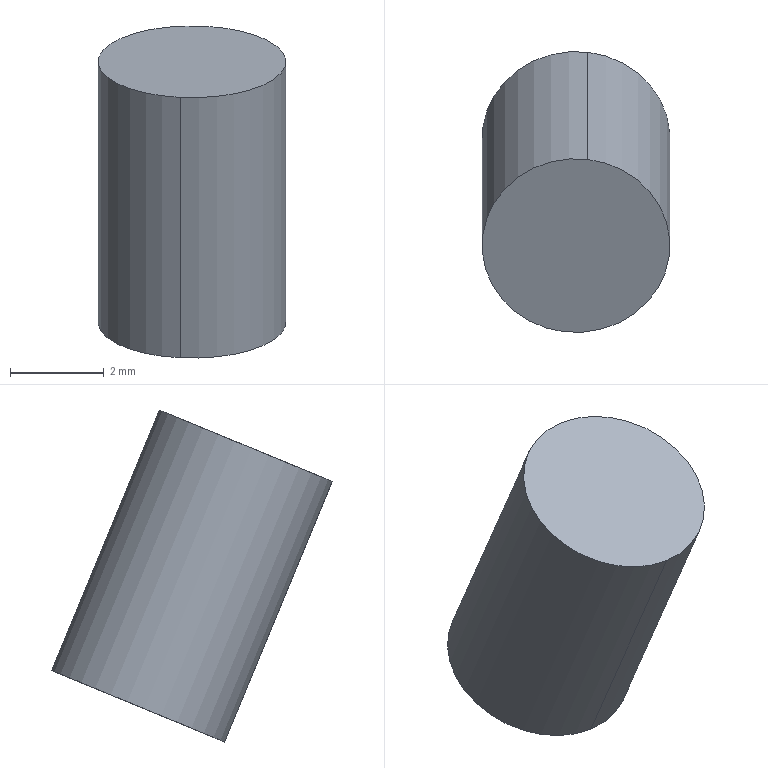Component | SolidWorks | Mirrorpin2-5 | 1 solid | 4 faces | box 4 x 5.99 x 7.07 mm | volume 75 mm3 | cylinder 2 | plane 2 | commonest cylinder face diameters 4 x2
STEP:
#1=COLOUR_RGB('',0.7922,0.8196,0.9333);
#2=FILL_AREA_STYLE_COLOUR('',#1);
#3=FILL_AREA_STYLE('',(#2));
#4=SURFACE_STYLE_FILL_AREA(#3);
#5=SURFACE_SIDE_STYLE('',(#4));
#6=SURFACE_STYLE_USAGE(.BOTH.,#5);
#7=PRESENTATION_STYLE_ASSIGNMENT((#6));
#8=CARTESIAN_POINT('',(13.341,-0.5746,2.179));
#9=VERTEX_POINT('',#8);
#10=CARTESIAN_POINT('',(13.322,-0.7191,2.119));
#11=VERTEX_POINT('',#10);
#12=CARTESIAN_POINT('',(13.332,-0.6469,2.149));
#13=DIRECTION('',(0.,-0.3818,0.9242));
#14=DIRECTION('',(-0.1245,-0.917,-0.3789));
#15=AXIS2_PLACEMENT_3D('',#12,#13,#14);
#16=CIRCLE('',#15,0.07874);
#17=EDGE_CURVE('',#9,#11,#16,.T.);
#18=ORIENTED_EDGE('',*,*,#17,.T.);
#19=CARTESIAN_POINT('',(13.322,-0.8093,2.337));
#20=VERTEX_POINT('',#19);
#21=CARTESIAN_POINT('',(13.322,-0.7191,2.119));
#22=DIRECTION('',(0.,-0.3818,0.9242));
#23=VECTOR('',#22,39.37);
#24=LINE('',#21,#23);
#25=EDGE_CURVE('',#11,#20,#24,.T.);
#26=ORIENTED_EDGE('',*,*,#25,.T.);
#27=CARTESIAN_POINT('',(13.341,-0.6648,2.397));
#28=VERTEX_POINT('',#27);
#29=CARTESIAN_POINT('',(13.332,-0.7371,2.367));
#30=DIRECTION('',(0.,-0.3818,0.9242));
#31=DIRECTION('',(-0.1245,-0.917,-0.3789));
#32=AXIS2_PLACEMENT_3D('',#29,#30,#31);
#33=CIRCLE('',#32,0.07874);
#34=EDGE_CURVE('',#28,#20,#33,.T.);
#35=ORIENTED_EDGE('',*,*,#34,.F.);
#36=CARTESIAN_POINT('',(13.341,-0.5746,2.179));
#37=DIRECTION('',(0.,-0.3818,0.9242));
#38=VECTOR('',#37,39.37);
#39=LINE('',#36,#38);
#40=EDGE_CURVE('',#9,#28,#39,.T.);
#41=ORIENTED_EDGE('',*,*,#40,.F.);
#42=EDGE_LOOP('',(#18,#26,#35,#41));
#43=FACE_OUTER_BOUND('',#42,.T.);
#44=CARTESIAN_POINT('',(13.332,-0.6469,2.149));
#45=DIRECTION('',(0.,-0.3818,0.9242));
#46=DIRECTION('',(0.1245,0.917,0.3789));
#47=AXIS2_PLACEMENT_3D('',#44,#45,#46);
#48=CYLINDRICAL_SURFACE('',#47,0.07874);
#49=ADVANCED_FACE('',(#43),#48,.T.);
#50=ORIENTED_EDGE('',*,*,#25,.F.);
#51=CARTESIAN_POINT('',(13.332,-0.6469,2.149));
#52=DIRECTION('',(0.,-0.3818,0.9242));
#53=DIRECTION('',(-0.1245,-0.917,-0.3789));
#54=AXIS2_PLACEMENT_3D('',#51,#52,#53);
#55=CIRCLE('',#54,0.07874);
#56=EDGE_CURVE('',#11,#9,#55,.T.);
#57=ORIENTED_EDGE('',*,*,#56,.T.);
#58=ORIENTED_EDGE('',*,*,#40,.T.);
#59=CARTESIAN_POINT('',(13.332,-0.7371,2.367));
#60=DIRECTION('',(0.,-0.3818,0.9242));
#61=DIRECTION('',(-0.1245,-0.917,-0.3789));
#62=AXIS2_PLACEMENT_3D('',#59,#60,#61);
#63=CIRCLE('',#62,0.07874);
#64=EDGE_CURVE('',#20,#28,#63,.T.);
#65=ORIENTED_EDGE('',*,*,#64,.F.);
#66=EDGE_LOOP('',(#50,#57,#58,#65));
#67=FACE_OUTER_BOUND('',#66,.T.);
#68=CARTESIAN_POINT('',(13.332,-0.6469,2.149));
#69=DIRECTION('',(0.,-0.3818,0.9242));
#70=DIRECTION('',(0.1245,0.917,0.3789));
#71=AXIS2_PLACEMENT_3D('',#68,#69,#70);
#72=CYLINDRICAL_SURFACE('',#71,0.07874);
#73=ADVANCED_FACE('',(#67),#72,.T.);
#74=ORIENTED_EDGE('',*,*,#17,.F.);
#75=ORIENTED_EDGE('',*,*,#56,.F.);
#76=EDGE_LOOP('',(#74,#75));
#77=FACE_OUTER_BOUND('',#76,.T.);
#78=CARTESIAN_POINT('',(13.332,-0.6469,2.149));
#79=DIRECTION('',(-0.,0.3818,-0.9242));
#80=DIRECTION('',(-0.1245,-0.917,-0.3789));
#81=AXIS2_PLACEMENT_3D('',#78,#79,#80);
#82=PLANE('',#81);
#83=ADVANCED_FACE('',(#77),#82,.T.);
#84=ORIENTED_EDGE('',*,*,#34,.T.);
#85=ORIENTED_EDGE('',*,*,#64,.T.);
#86=EDGE_LOOP('',(#84,#85));
#87=FACE_OUTER_BOUND('',#86,.T.);
#88=CARTESIAN_POINT('',(13.332,-0.7371,2.367));
#89=DIRECTION('',(-0.,0.3818,-0.9242));
#90=DIRECTION('',(-0.1245,-0.917,-0.3789));
#91=AXIS2_PLACEMENT_3D('',#88,#89,#90);
#92=PLANE('',#91);
#93=ADVANCED_FACE('',(#87),#92,.F.);
#94=CLOSED_SHELL('',(#49,#73,#83,#93));
#95=MANIFOLD_SOLID_BREP('',#94);
#96=STYLED_ITEM('',(#7),#95);
#97=(LENGTH_UNIT()NAMED_UNIT(*)SI_UNIT($,.METRE.));
#98=LENGTH_MEASURE_WITH_UNIT(LENGTH_MEASURE(0.0254),#97);
#99=DIMENSIONAL_EXPONENTS(1.,0.,0.,0.,0.,0.,0.);
#100=(CONVERSION_BASED_UNIT('',#98)LENGTH_UNIT()NAMED_UNIT(#99));
#101=UNCERTAINTY_MEASURE_WITH_UNIT(LENGTH_MEASURE(0.00001),#100,'','');
#102=(NAMED_UNIT(*)PLANE_ANGLE_UNIT()SI_UNIT($,.RADIAN.));
#103=(NAMED_UNIT(*)SI_UNIT($,.STERADIAN.)SOLID_ANGLE_UNIT());
#104=(GEOMETRIC_REPRESENTATION_CONTEXT(3)GLOBAL_UNCERTAINTY_ASSIGNED_CONTEXT((#101))GLOBAL_UNIT_ASSIGNED_CONTEXT((#100,#102,#103))REPRESENTATION_CONTEXT('',''));
#105=MECHANICAL_DESIGN_GEOMETRIC_PRESENTATION_REPRESENTATION('',(#96),#104);
#106=CARTESIAN_POINT('',(0.,0.,0.));
#107=DIRECTION('',(0.,0.,1.));
#108=DIRECTION('',(1.,0.,0.));
#109=AXIS2_PLACEMENT_3D('',#106,#107,#108);
#110=(LENGTH_UNIT()NAMED_UNIT(*)SI_UNIT($,.METRE.));
#111=LENGTH_MEASURE_WITH_UNIT(LENGTH_MEASURE(0.0254),#110);
#112=DIMENSIONAL_EXPONENTS(1.,0.,0.,0.,0.,0.,0.);
#113=(CONVERSION_BASED_UNIT('',#111)LENGTH_UNIT()NAMED_UNIT(#112));
#114=UNCERTAINTY_MEASURE_WITH_UNIT(LENGTH_MEASURE(0.00001),#113,'','');
#115=(NAMED_UNIT(*)PLANE_ANGLE_UNIT()SI_UNIT($,.RADIAN.));
#116=(NAMED_UNIT(*)SI_UNIT($,.STERADIAN.)SOLID_ANGLE_UNIT());
#117=(GEOMETRIC_REPRESENTATION_CONTEXT(3)GLOBAL_UNCERTAINTY_ASSIGNED_CONTEXT((#114))GLOBAL_UNIT_ASSIGNED_CONTEXT((#113,#115,#116))REPRESENTATION_CONTEXT('',''));
#118=ADVANCED_BREP_SHAPE_REPRESENTATION('',(#95,#109),#117);
#119=PRESENTATION_LAYER_ASSIGNMENT('','',(#96));